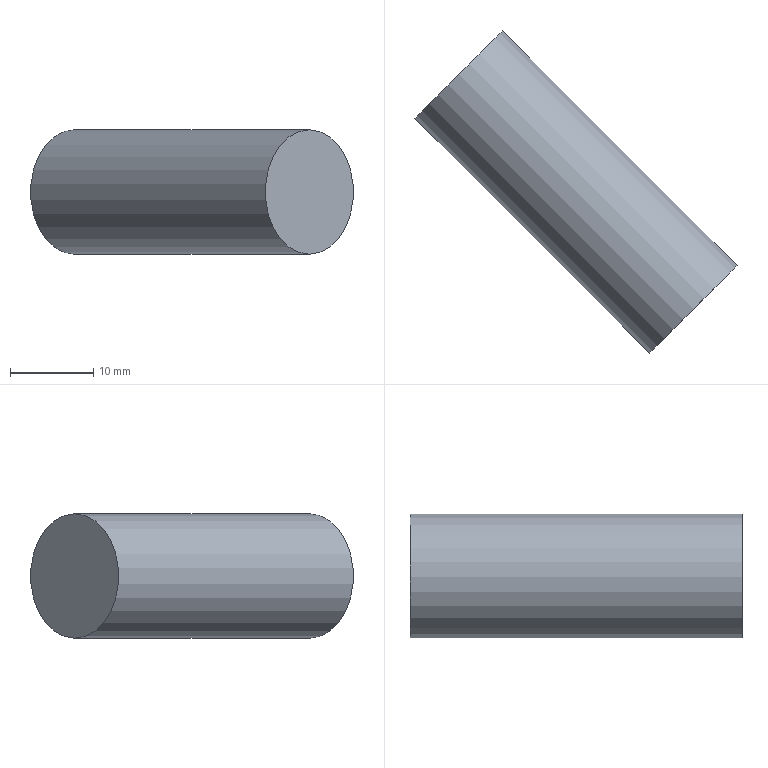Component | NX | SLIDER_FRAME_PIN_2 | 1 solid | 3 faces | box 38.89 x 38.89 x 15 mm | volume 7069 mm3 | plane 2 | cylinder 1 | commonest cylinder face diameters 15 x1
STEP:
#1=CARTESIAN_POINT('',(0.,0.,0.));
#2=DIRECTION('',(0.,0.,1.));
#3=DIRECTION('',(1.,0.,0.));
#4=AXIS2_PLACEMENT_3D('',#1,#2,#3);
#5=CARTESIAN_POINT('',(-579.895,703.013,-627.5));
#6=VERTEX_POINT('',#5);
#7=CARTESIAN_POINT('',(-579.895,703.013,-620.));
#8=DIRECTION('',(0.7071,-0.7071,0.));
#9=DIRECTION('',(0.,0.,-1.));
#10=AXIS2_PLACEMENT_3D('',#7,#8,#9);
#11=CIRCLE('',#10,7.5);
#12=CARTESIAN_POINT('',(-579.895,703.013,-620.));
#13=DIRECTION('',(-0.7071,0.7071,0.));
#14=DIRECTION('',(0.,0.,-1.));
#15=AXIS2_PLACEMENT_3D('',#12,#13,#14);
#16=PLANE('',#15);
#17=CARTESIAN_POINT('',(7.5,0.));
#18=CARTESIAN_POINT('',(7.5,-12.99));
#19=CARTESIAN_POINT('',(-3.75,-6.495));
#20=CARTESIAN_POINT('',(-15.,-0.));
#21=CARTESIAN_POINT('',(-3.75,6.495));
#22=CARTESIAN_POINT('',(7.5,12.99));
#23=CARTESIAN_POINT('',(7.5,0.));
#24=(BOUNDED_CURVE()B_SPLINE_CURVE(2,(#17,#18,#19,#20,#21,#22,#23),.UNSPECIFIED.,.T.,.F.)B_SPLINE_CURVE_WITH_KNOTS((1,2,2,2,2,1),(-2.094,0.,2.094,4.189,6.283,8.378),.UNSPECIFIED.)CURVE()GEOMETRIC_REPRESENTATION_ITEM()RATIONAL_B_SPLINE_CURVE((1.,0.5,1.,0.5,1.,0.5,1.))REPRESENTATION_ITEM(''));
#25=(GEOMETRIC_REPRESENTATION_CONTEXT(2)PARAMETRIC_REPRESENTATION_CONTEXT()REPRESENTATION_CONTEXT('',''));
#26=DEFINITIONAL_REPRESENTATION('',(#24),#25);
#27=PCURVE('',#16,#26);
#28=CARTESIAN_POINT('',(-551.611,674.729,-620.));
#29=DIRECTION('',(-0.7071,0.7071,0.));
#30=DIRECTION('',(0.,0.,-1.));
#31=AXIS2_PLACEMENT_3D('',#28,#29,#30);
#32=CYLINDRICAL_SURFACE('',#31,7.5);
#33=CARTESIAN_POINT('',(6.283,40.));
#34=DIRECTION('',(-1.,0.));
#35=VECTOR('',#34,1.);
#36=LINE('',#33,#35);
#37=(GEOMETRIC_REPRESENTATION_CONTEXT(2)PARAMETRIC_REPRESENTATION_CONTEXT()REPRESENTATION_CONTEXT('',''));
#38=DEFINITIONAL_REPRESENTATION('',(#36),#37);
#39=PCURVE('',#32,#38);
#40=SURFACE_CURVE('',#11,(#27,#39),.PCURVE_S1.);
#41=EDGE_CURVE('',#6,#6,#40,.T.);
#42=ORIENTED_EDGE('',*,*,#41,.F.);
#43=EDGE_LOOP('',(#42));
#44=FACE_BOUND('',#43,.T.);
#45=ADVANCED_FACE('',(#44),#16,.T.);
#46=CARTESIAN_POINT('',(-551.611,674.729,-627.5));
#47=VERTEX_POINT('',#46);
#48=CARTESIAN_POINT('',(-551.611,674.729,-620.));
#49=DIRECTION('',(-0.7071,0.7071,0.));
#50=DIRECTION('',(0.,0.,-1.));
#51=AXIS2_PLACEMENT_3D('',#48,#49,#50);
#52=CIRCLE('',#51,7.5);
#53=CARTESIAN_POINT('',(-551.611,674.729,-620.));
#54=DIRECTION('',(0.7071,-0.7071,0.));
#55=DIRECTION('',(0.,0.,1.));
#56=AXIS2_PLACEMENT_3D('',#53,#54,#55);
#57=PLANE('',#56);
#58=CARTESIAN_POINT('',(-7.5,0.));
#59=CARTESIAN_POINT('',(-7.5,12.99));
#60=CARTESIAN_POINT('',(3.75,6.495));
#61=CARTESIAN_POINT('',(15.,0.));
#62=CARTESIAN_POINT('',(3.75,-6.495));
#63=CARTESIAN_POINT('',(-7.5,-12.99));
#64=CARTESIAN_POINT('',(-7.5,0.));
#65=(BOUNDED_CURVE()B_SPLINE_CURVE(2,(#58,#59,#60,#61,#62,#63,#64),.UNSPECIFIED.,.T.,.F.)B_SPLINE_CURVE_WITH_KNOTS((1,2,2,2,2,1),(-2.094,0.,2.094,4.189,6.283,8.378),.UNSPECIFIED.)CURVE()GEOMETRIC_REPRESENTATION_ITEM()RATIONAL_B_SPLINE_CURVE((1.,0.5,1.,0.5,1.,0.5,1.))REPRESENTATION_ITEM(''));
#66=(GEOMETRIC_REPRESENTATION_CONTEXT(2)PARAMETRIC_REPRESENTATION_CONTEXT()REPRESENTATION_CONTEXT('',''));
#67=DEFINITIONAL_REPRESENTATION('',(#65),#66);
#68=PCURVE('',#57,#67);
#69=CARTESIAN_POINT('',(0.,0.));
#70=DIRECTION('',(1.,0.));
#71=VECTOR('',#70,1.);
#72=LINE('',#69,#71);
#73=(GEOMETRIC_REPRESENTATION_CONTEXT(2)PARAMETRIC_REPRESENTATION_CONTEXT()REPRESENTATION_CONTEXT('',''));
#74=DEFINITIONAL_REPRESENTATION('',(#72),#73);
#75=PCURVE('',#32,#74);
#76=SURFACE_CURVE('',#52,(#68,#75),.PCURVE_S1.);
#77=EDGE_CURVE('',#47,#47,#76,.T.);
#78=ORIENTED_EDGE('',*,*,#77,.F.);
#79=EDGE_LOOP('',(#78));
#80=FACE_BOUND('',#79,.T.);
#81=ADVANCED_FACE('',(#80),#57,.T.);
#82=ORIENTED_EDGE('',*,*,#41,.T.);
#83=CARTESIAN_POINT('',(-551.611,674.729,-627.5));
#84=CARTESIAN_POINT('',(-579.895,703.013,-627.5));
#85=B_SPLINE_CURVE_WITH_KNOTS('',1,(#83,#84),.UNSPECIFIED.,.F.,.F.,(2,2),(0.,40.),.PIECEWISE_BEZIER_KNOTS.);
#86=CARTESIAN_POINT('',(0.,0.));
#87=DIRECTION('',(0.,1.));
#88=VECTOR('',#87,1.);
#89=LINE('',#86,#88);
#90=(GEOMETRIC_REPRESENTATION_CONTEXT(2)PARAMETRIC_REPRESENTATION_CONTEXT()REPRESENTATION_CONTEXT('',''));
#91=DEFINITIONAL_REPRESENTATION('',(#89),#90);
#92=PCURVE('',#32,#91);
#93=CARTESIAN_POINT('',(6.283,0.));
#94=DIRECTION('',(0.,1.));
#95=VECTOR('',#94,1.);
#96=LINE('',#93,#95);
#97=(GEOMETRIC_REPRESENTATION_CONTEXT(2)PARAMETRIC_REPRESENTATION_CONTEXT()REPRESENTATION_CONTEXT('',''));
#98=DEFINITIONAL_REPRESENTATION('',(#96),#97);
#99=PCURVE('',#32,#98);
#100=SEAM_CURVE('',#85,(#92,#99),.PCURVE_S1.);
#101=EDGE_CURVE('',#47,#6,#100,.T.);
#102=ORIENTED_EDGE('',*,*,#101,.F.);
#103=ORIENTED_EDGE('',*,*,#77,.T.);
#104=ORIENTED_EDGE('',*,*,#101,.T.);
#105=EDGE_LOOP('',(#82,#102,#103,#104));
#106=FACE_BOUND('',#105,.T.);
#107=ADVANCED_FACE('',(#106),#32,.T.);
#108=CLOSED_SHELL('',(#45,#81,#107));
#109=MANIFOLD_SOLID_BREP('',#108);
#110=(LENGTH_UNIT()NAMED_UNIT(*)SI_UNIT(.MILLI.,.METRE.));
#111=UNCERTAINTY_MEASURE_WITH_UNIT(LENGTH_MEASURE(0.00001),#110,'','');
#112=(NAMED_UNIT(*)PLANE_ANGLE_UNIT()SI_UNIT($,.RADIAN.));
#113=(NAMED_UNIT(*)SI_UNIT($,.STERADIAN.)SOLID_ANGLE_UNIT());
#114=(GEOMETRIC_REPRESENTATION_CONTEXT(3)GLOBAL_UNCERTAINTY_ASSIGNED_CONTEXT((#111))GLOBAL_UNIT_ASSIGNED_CONTEXT((#110,#112,#113))REPRESENTATION_CONTEXT('',''));
#115=ADVANCED_BREP_SHAPE_REPRESENTATION('',(#4,#109),#114);